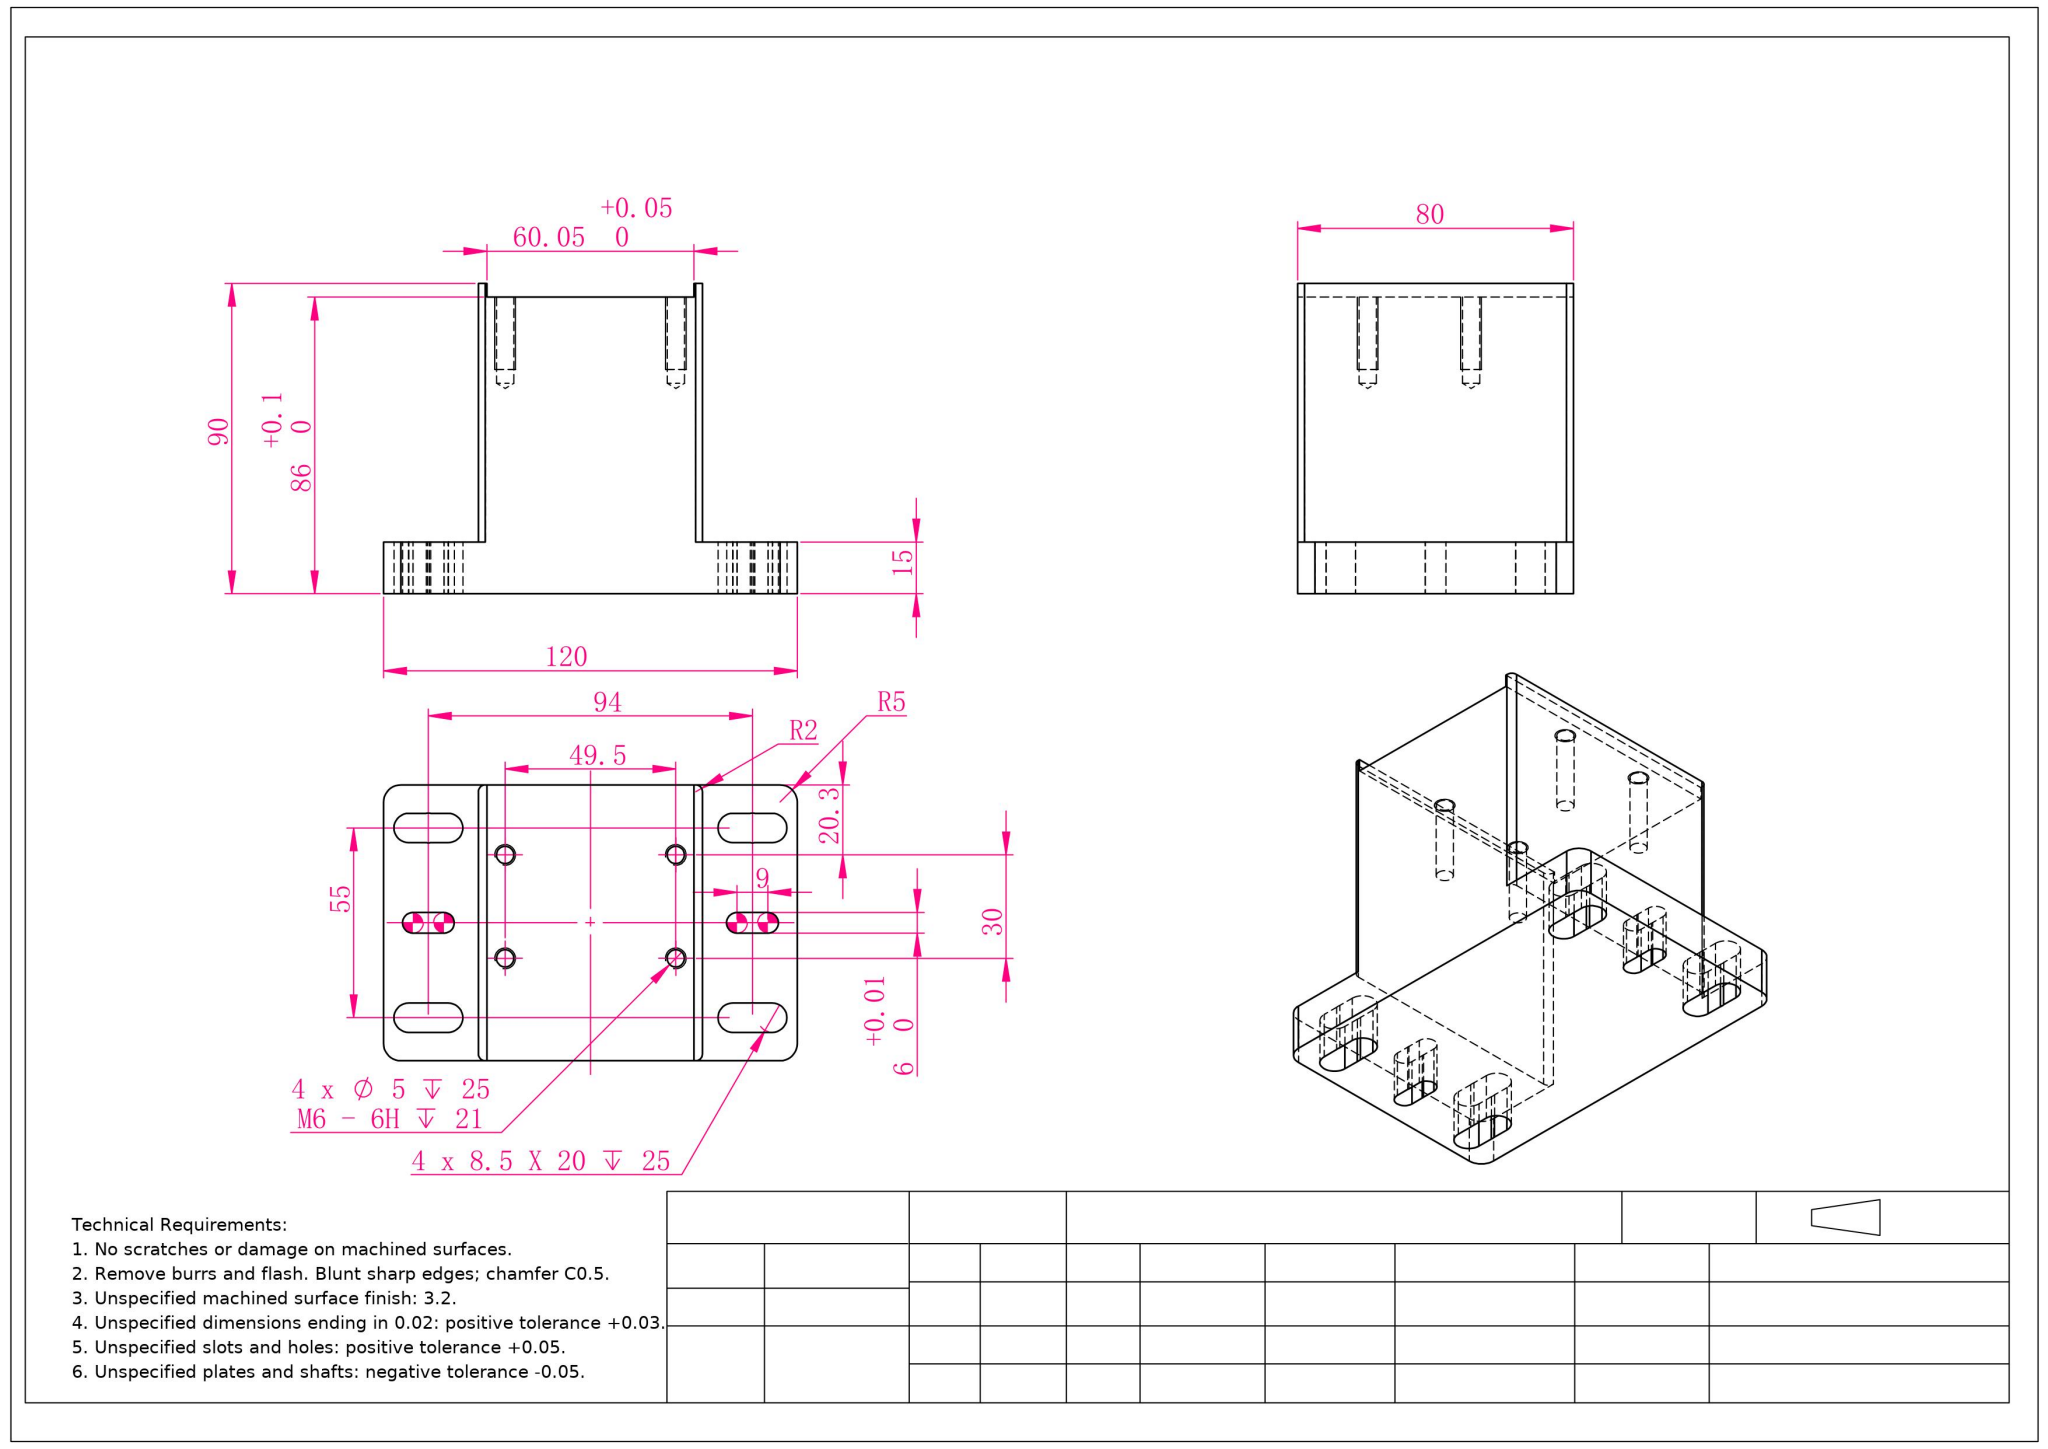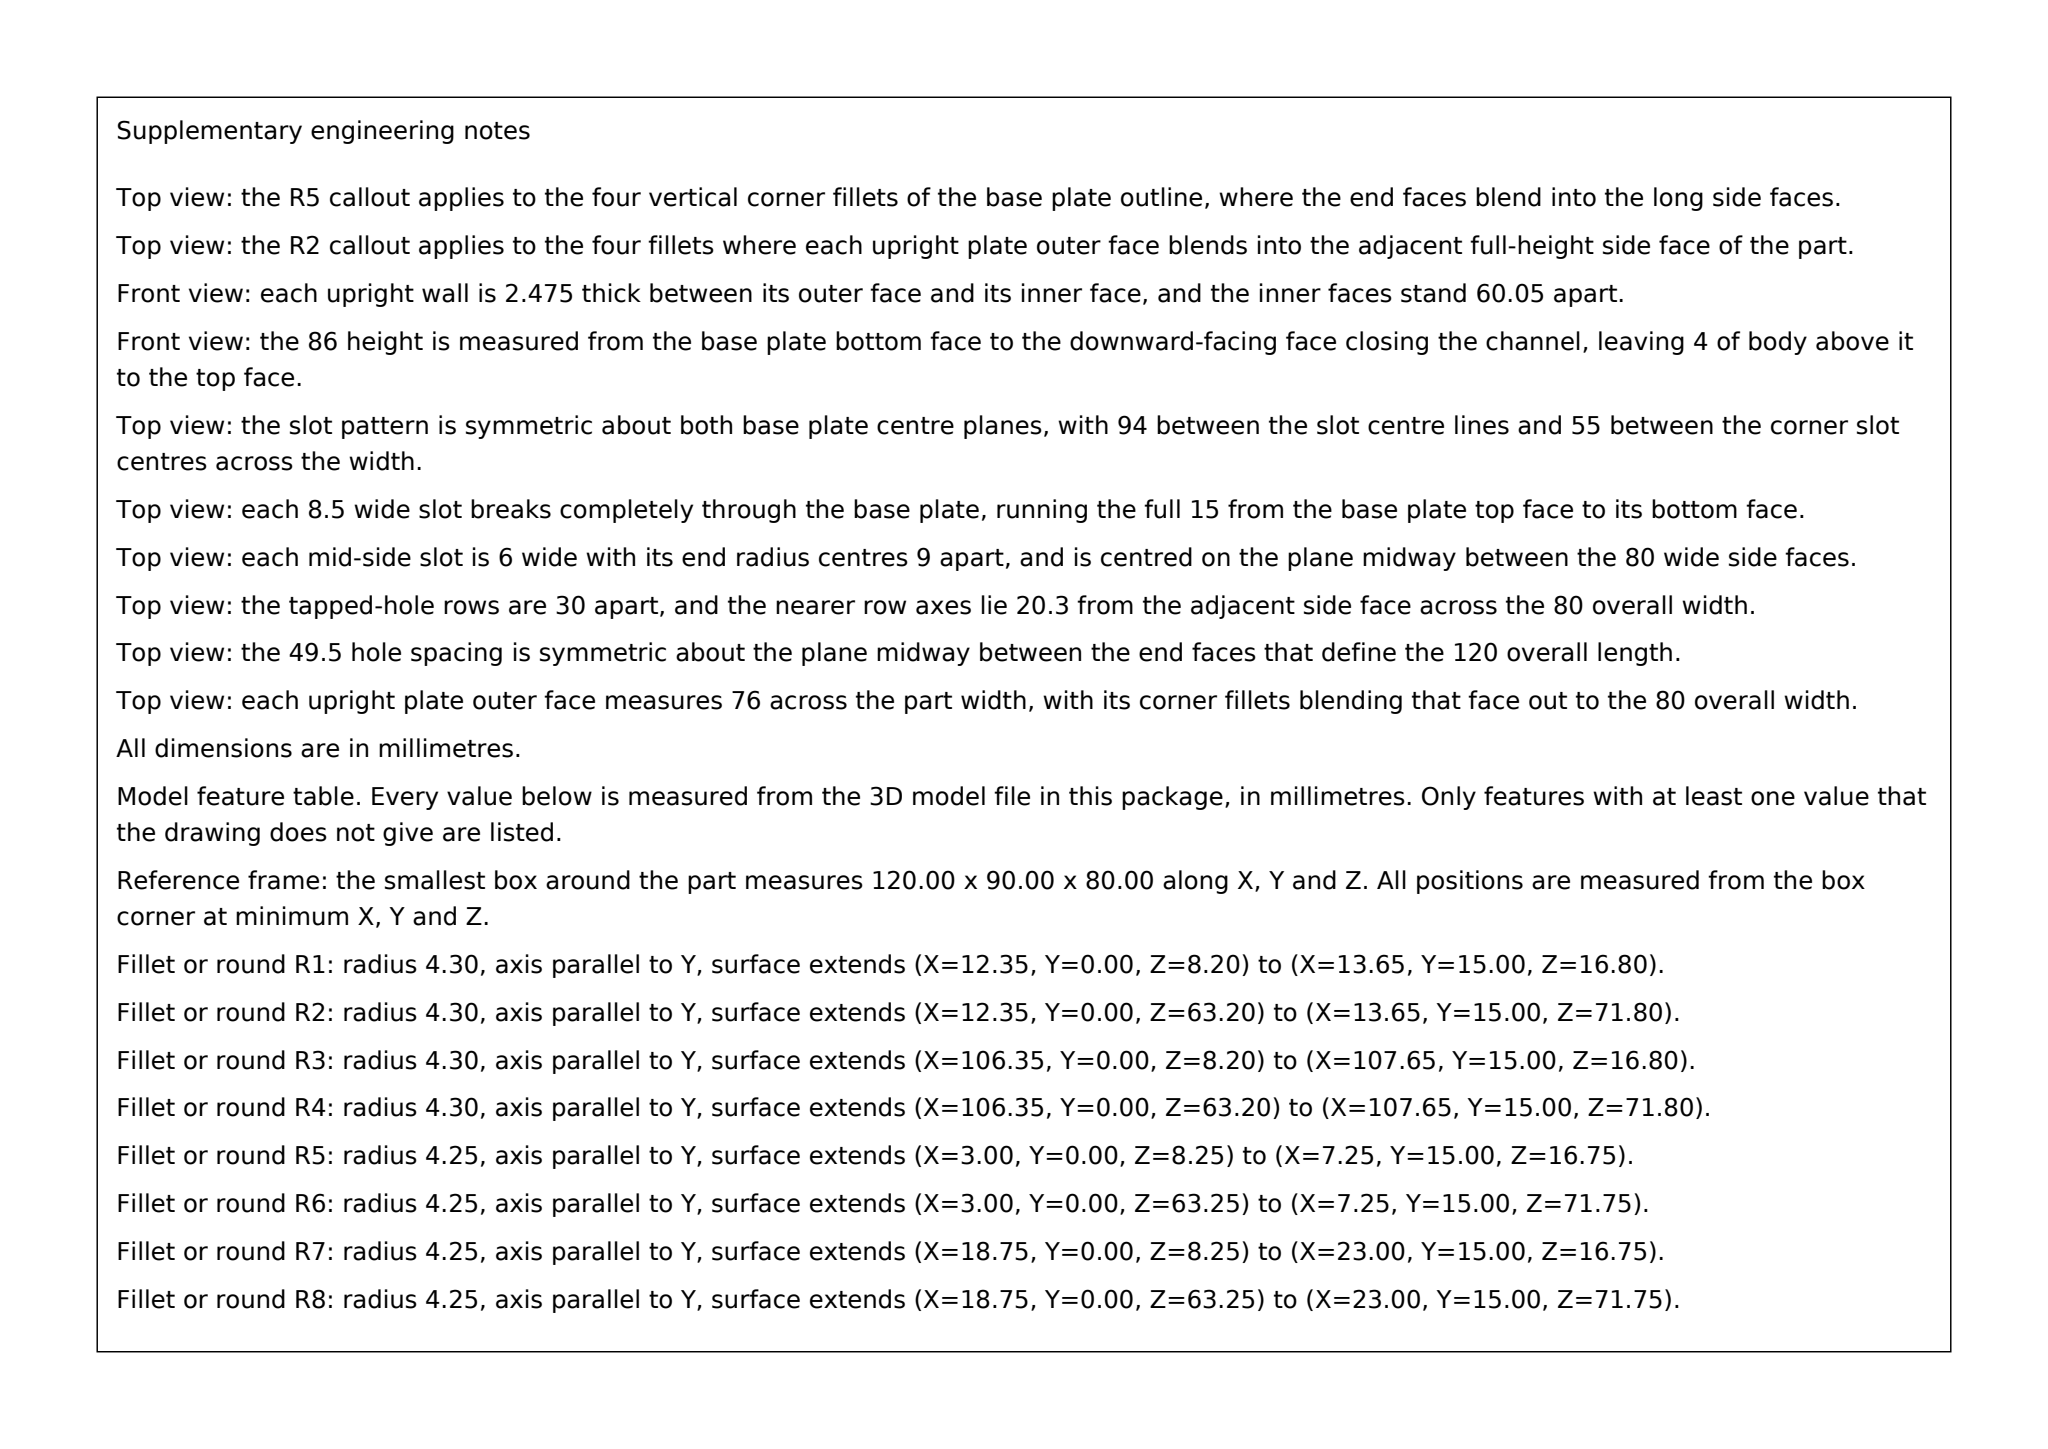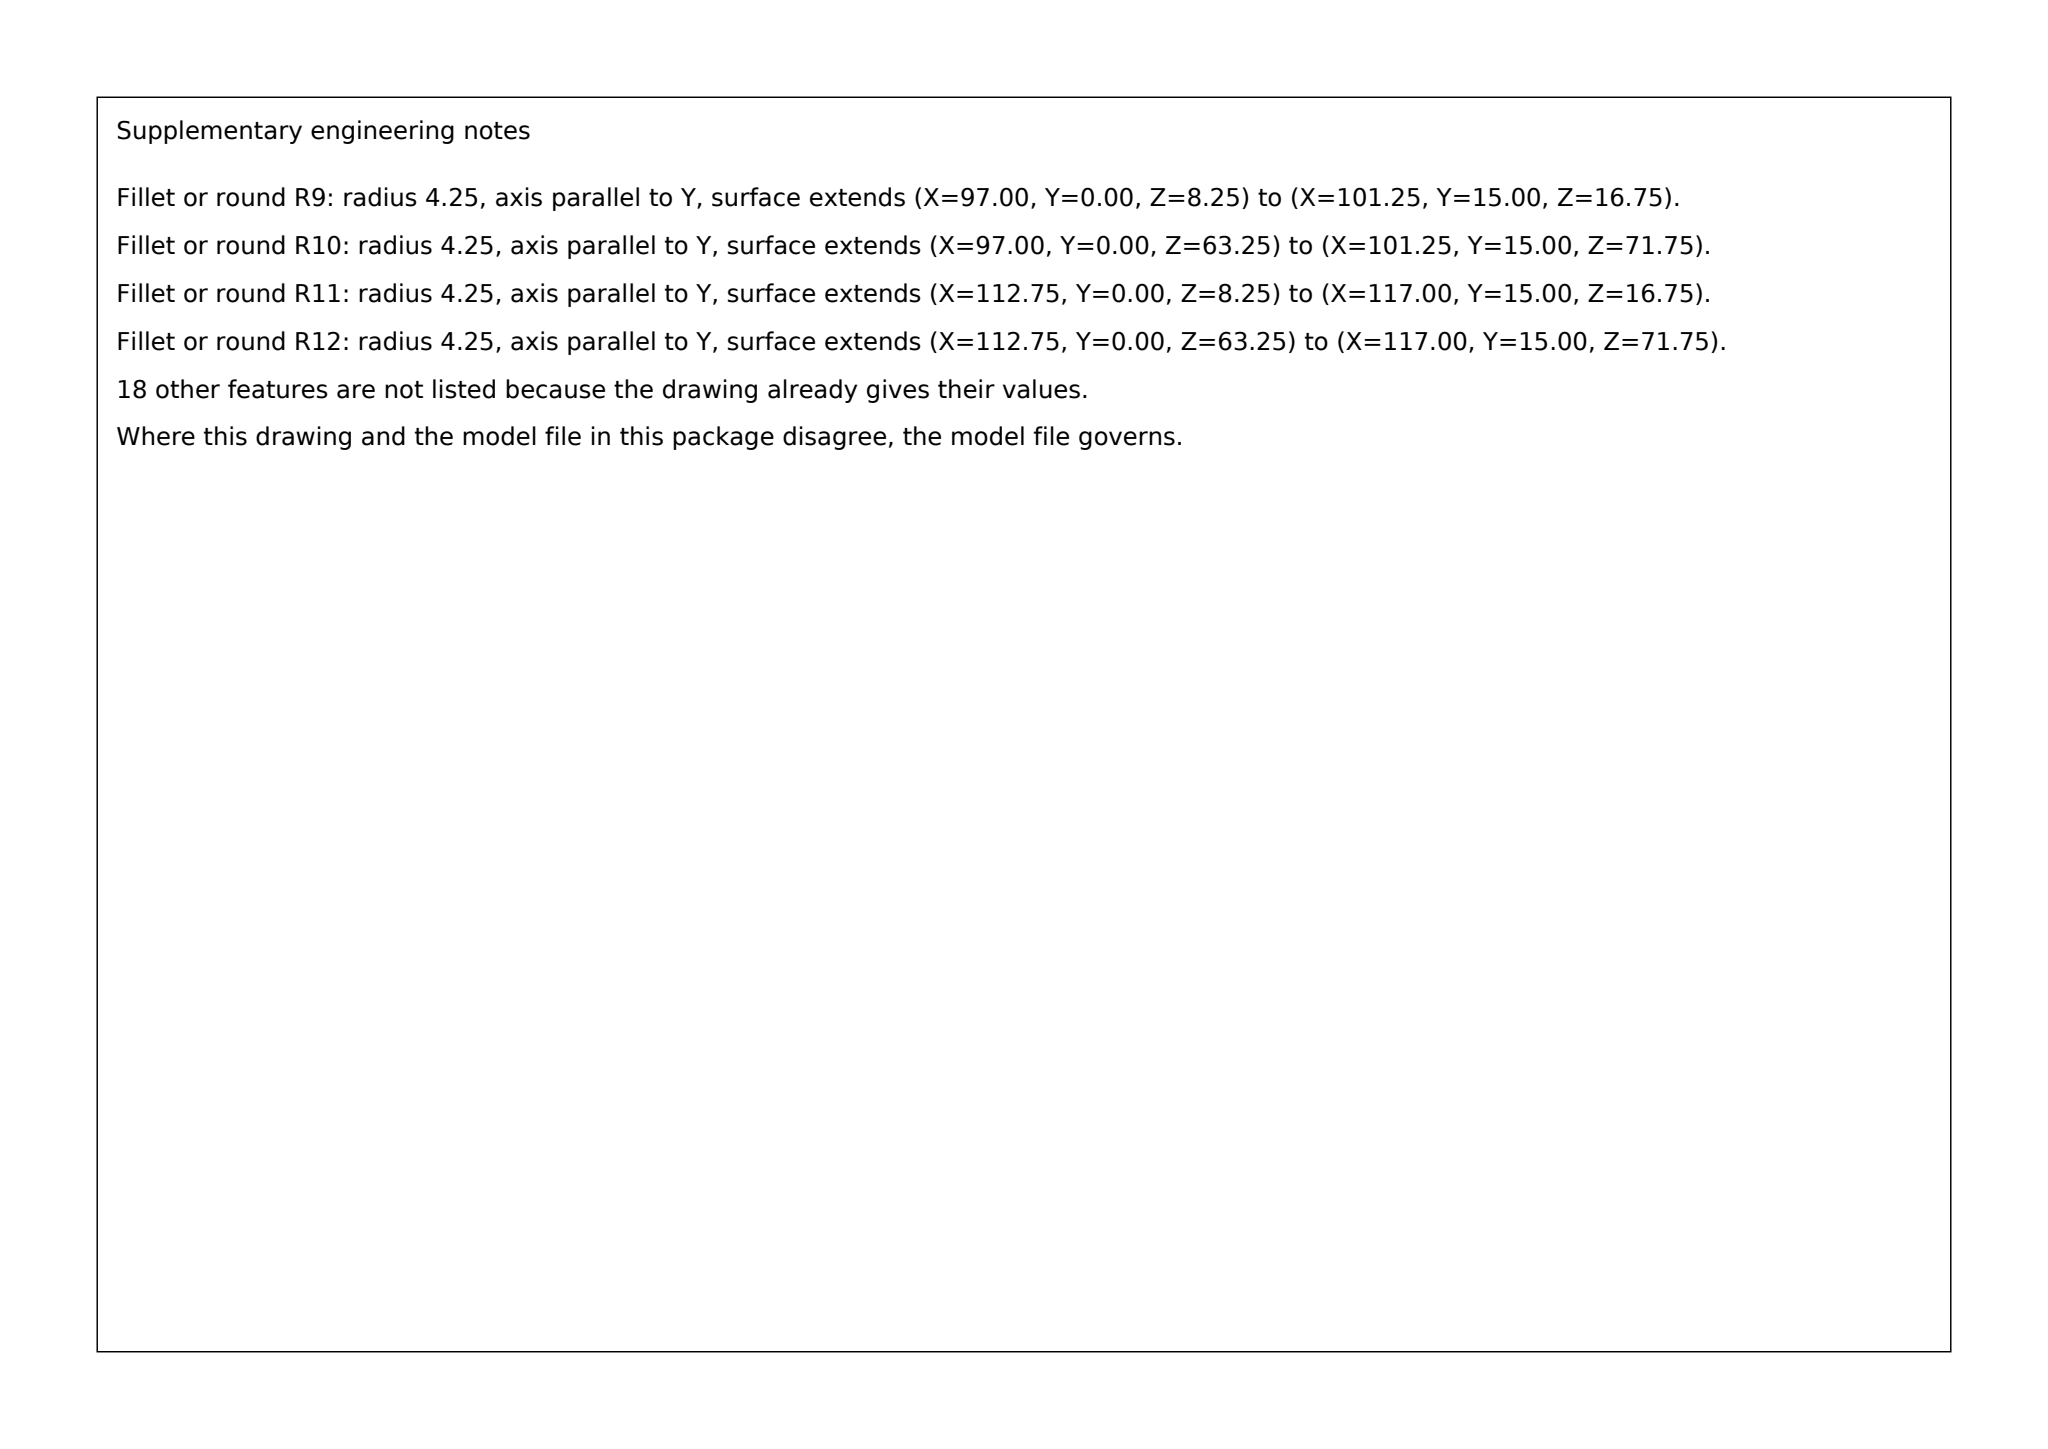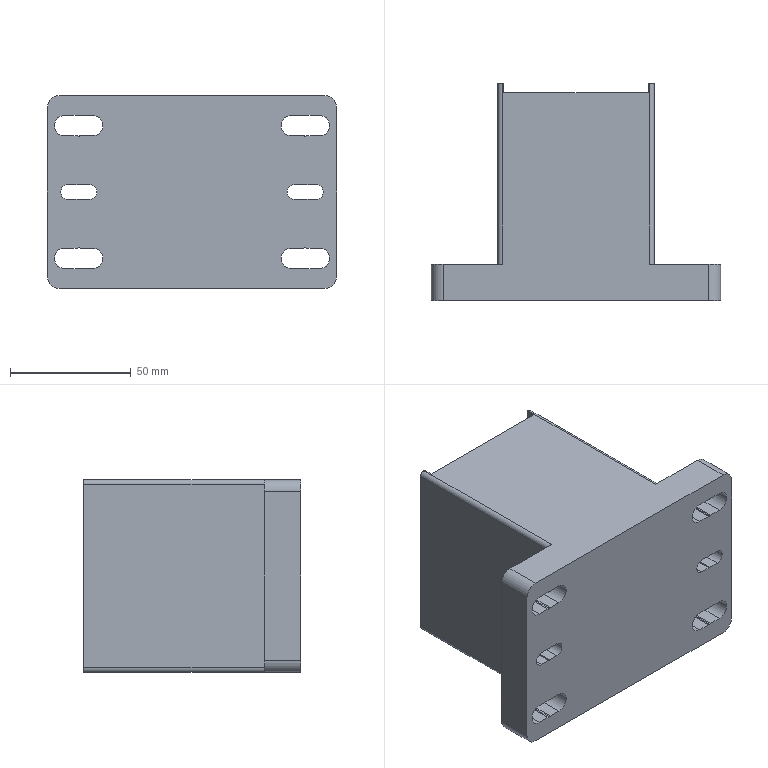Part | SolidWorks | mm | material 6061 Aluminum Oxide | 1 solid | 92 faces | box 120 x 90 x 80 mm | volume 500458 mm3 | cylinder 46 | plane 38 | cone 8 | commonest cylinder face diameters 8.6 x12 5 x8 8.5 x8 6.02 x6 10 x4 6 x4 4 x4
Drawing notes:
VERT PLATES 2.5 THK, 2 PL | from the solid: Vertical plate faces at x=27.5 and x=30.0 (and x=90.0 and x=92.5), extents y[15,90]/y[86,90] -> plate thickness 2.5 mm, 2 places
FRONT VIEW DASHED FEAT = 4X Ø5 DP 25 FROM 86 FACE, 49.5 X 30 CTRS | from the solid: hole/bore Ø5, axis y, at x=35.3 & 84.8, z=20.3 & 50.3, from y61 to y86 (25 deep below the y=86 face); spacing 49.5 in X, 30 in Z
GARBLED LEADER = 65 O/A WIDTH ACROSS UPRIGHTS, 2.5 THK EA | from the solid: x-planes at 27.5 and 92.5 (y15-90) give 65 outside width; inner faces x=30 & 90 (60.05 dim) give 2.5 wall thk